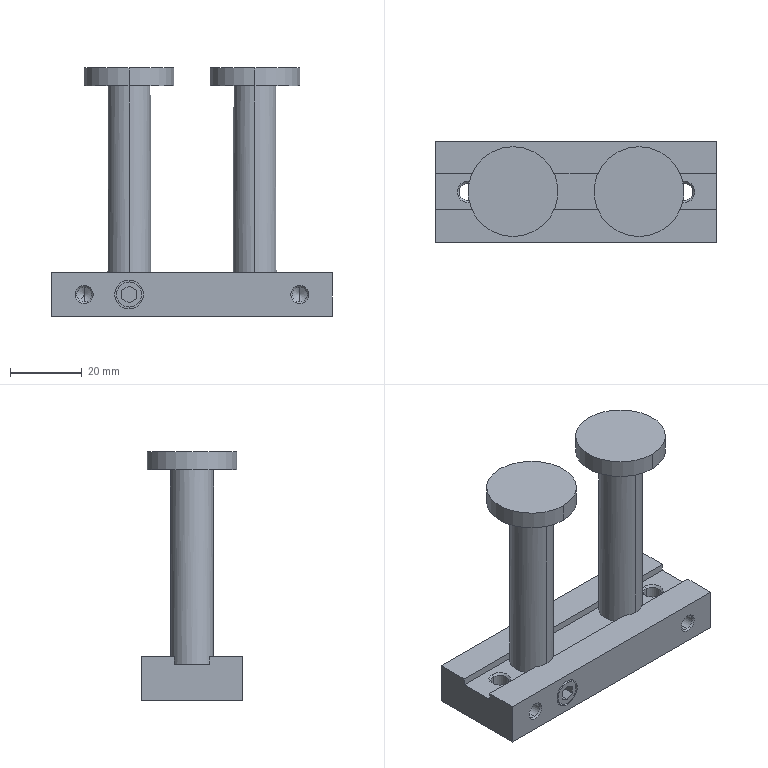Component | SolidWorks | CXSM25-10-Z73(0_0_0)-2_CXSM25-10(0_0)_ROD-1 | 1 solid | 90 faces | box 78 x 28 x 69 mm | volume 40711 mm3 | plane 38 | cylinder 28 | cone 24 | commonest cylinder face diameters 4.134 x8 4.917 x4 25 x4 12 x4 7 x2 8 x2 10 x2 11 x2
build123d program:
from build123d import *

# Parameters (mm, degrees)
SKETCH1_W           = 28
SKETCH1_H           = 78
BOSS_EXTRUDE1_DEPTH = 12
SKETCH2_W           = 10
SKETCH2_H           = 78
CUT_EXTRUDE1_DEPTH  = 2
SKETCH11_R          = 5.5
SKETCH11_R_2        = 5
CUT_EXTRUDE2_DEPTH  = 1
CUT_EXTRUDE3_DEPTH  = 5.2
SKETCH13_R          = 4
SKETCH13_R_2        = 3.5
CUT_EXTRUDE4_DEPTH  = 1
CUT_EXTRUDE5_DEPTH  = 4


with BuildPart() as part:
    # Sketch1 → Boss-Extrude1 (new body)
    with BuildSketch(Plane.XY.offset(12)):
        Rectangle(SKETCH1_W, SKETCH1_H)
    extrude(amount=BOSS_EXTRUDE1_DEPTH)

    # Sketch2 → Cut-Extrude1 (cut)
    with BuildSketch(Plane.XY.offset(12)):
        Rectangle(SKETCH2_W, SKETCH2_H)
    extrude(amount=CUT_EXTRUDE1_DEPTH, mode=Mode.SUBTRACT)

    # Sketch3 → Revolve1 (revolve)
    with BuildSketch(Plane(origin=(0, 0, 0), x_dir=(0, 0, -1), z_dir=(1, 0, 0)), mode=Mode.PRIVATE) as revolve1_sk:
        Polygon((-17, 17.5), (-17, 23.5), (40, 23.5), (40, 30), (45, 30), (45, 17.5), align=None)
    revolve(revolve1_sk.sketch.rotate(Axis((0, 17.5, -45), (0, 0, 1)), 270), axis=Axis((0, 17.5, -45), (0, 0, 1)))

    # Sketch4 → Revolve2 (revolve)
    with BuildSketch(Plane(origin=(0, 0, 0), x_dir=(0, 0, -1), z_dir=(1, 0, 0)), mode=Mode.PRIVATE) as revolve2_sk:
        Polygon((-17, -17.5), (-17, -11.5), (40, -11.5), (40, -5), (45, -5), (45, -17.5), align=None)
    revolve(revolve2_sk.sketch.rotate(Axis((0, -17.5, -45), (0, 0, 1)), 270), axis=Axis((0, -17.5, -45), (0, 0, 1)))

    # Sketch5 → Cut-Revolve1 (revolve, cut)
    with BuildSketch(Plane(origin=(0, 0, 0), x_dir=(0, 0, -1), z_dir=(1, 0, 0)), mode=Mode.PRIVATE) as cut_revolve1_sk:
        Polygon((-24, 30), (-24, 33), (-23.459, 32.459), (-14.541, 32.459), (-14, 33), (-14, 30), align=None)
    revolve(cut_revolve1_sk.sketch.rotate(Axis((0, 30, 14), (0, 0, 1)), 270), axis=Axis((0, 30, 14), (0, 0, 1)), mode=Mode.SUBTRACT)

    # Sketch6 → Cut-Revolve2 (revolve, cut)
    with BuildSketch(Plane(origin=(0, 0, 0), x_dir=(0, 0, -1), z_dir=(1, 0, 0)), mode=Mode.PRIVATE) as cut_revolve2_sk:
        Polygon((-24, -30), (-24, -27), (-23.459, -27.541), (-14.541, -27.541), (-14, -27), (-14, -30), align=None)
    revolve(cut_revolve2_sk.sketch.rotate(Axis((0, -30, 14), (0, 0, 1)), 270), axis=Axis((0, -30, 14), (0, 0, 1)), mode=Mode.SUBTRACT)

    # Sketch7 → Cut-Revolve3 (revolve, cut)
    with BuildSketch(Plane.XY.offset(18), mode=Mode.PRIVATE) as cut_revolve3_sk:
        Polygon((-14, 30), (-14, 32.5), (-13.567, 32.067), (-6.5, 32.067), (-5.307, 30), align=None)
    revolve(cut_revolve3_sk.sketch.rotate(Axis((-5.307, 30, 18), (-1, 0, 0)), 270), axis=Axis((-5.307, 30, 18), (-1, 0, 0)), mode=Mode.SUBTRACT)

    # Sketch8 → Cut-Revolve4 (revolve, cut)
    with BuildSketch(Plane.XY.offset(18), mode=Mode.PRIVATE) as cut_revolve4_sk:
        Polygon((-5.307, -30), (-6.5, -32.067), (-13.567, -32.067), (-14, -32.5), (-14, -30), align=None)
    revolve(cut_revolve4_sk.sketch.rotate(Axis((-14, -30, 18), (1, 0, 0)), 90), axis=Axis((-14, -30, 18), (1, 0, 0)), mode=Mode.SUBTRACT)

    # Sketch9 → Cut-Revolve5 (revolve, cut)
    with BuildSketch(Plane.XY.offset(18), mode=Mode.PRIVATE) as cut_revolve5_sk:
        Polygon((5.307, 30), (6.5, 32.067), (13.567, 32.067), (14, 32.5), (14, 30), align=None)
    revolve(cut_revolve5_sk.sketch.rotate(Axis((14, 30, 18), (-1, 0, 0)), 270), axis=Axis((14, 30, 18), (-1, 0, 0)), mode=Mode.SUBTRACT)

    # Sketch10 → Cut-Revolve6 (revolve, cut)
    with BuildSketch(Plane.XY.offset(18), mode=Mode.PRIVATE) as cut_revolve6_sk:
        Polygon((14, -30), (14, -32.5), (13.567, -32.067), (6.5, -32.067), (5.307, -30), align=None)
    revolve(cut_revolve6_sk.sketch.rotate(Axis((5.307, -30, 18), (1, 0, 0)), 90), axis=Axis((5.307, -30, 18), (1, 0, 0)), mode=Mode.SUBTRACT)

    # Sketch11 → Cut-Extrude2 (cut)
    with BuildSketch(Plane.XY.offset(24)):
        with Locations((0, -17.5)):
            Circle(SKETCH11_R)
        with Locations((0, -17.5)):
            Circle(SKETCH11_R_2, mode=Mode.SUBTRACT)
    extrude(amount=-CUT_EXTRUDE2_DEPTH, mode=Mode.SUBTRACT)

    # Sketch12 → Cut-Extrude3 (cut)
    with BuildSketch(Plane.XY.offset(24)):
        Polygon((-3.002, -17.5), (-1.501, -20.1), (1.501, -20.1), (3.002, -17.5), (1.501, -14.9), (-1.501, -14.9), align=None)
    extrude(amount=-CUT_EXTRUDE3_DEPTH, mode=Mode.SUBTRACT)

    # Sketch13 → Cut-Extrude4 (cut)
    with BuildSketch(Plane(origin=(14, 0, 0), x_dir=(0, 0, -1), z_dir=(1, 0, 0))):
        with Locations((-18, 17.5)):
            Circle(SKETCH13_R)
        with Locations((-18, 17.5)):
            Circle(SKETCH13_R_2, mode=Mode.SUBTRACT)
    extrude(amount=-CUT_EXTRUDE4_DEPTH, mode=Mode.SUBTRACT)

    # Sketch14 → Cut-Extrude5 (cut)
    with BuildSketch(Plane(origin=(14, 0, 0), x_dir=(0, 0, -1), z_dir=(1, 0, 0))):
        Polygon((-20.309, 17.5), (-19.155, 15.5), (-16.845, 15.5), (-15.691, 17.5), (-16.845, 19.5), (-19.155, 19.5), align=None)
    extrude(amount=-CUT_EXTRUDE5_DEPTH, mode=Mode.SUBTRACT)


solid = part.part

# Placed as in the assembly
solid = solid.moved(Location((955.266, 376.143, -256.265), (180, 0, 90)))